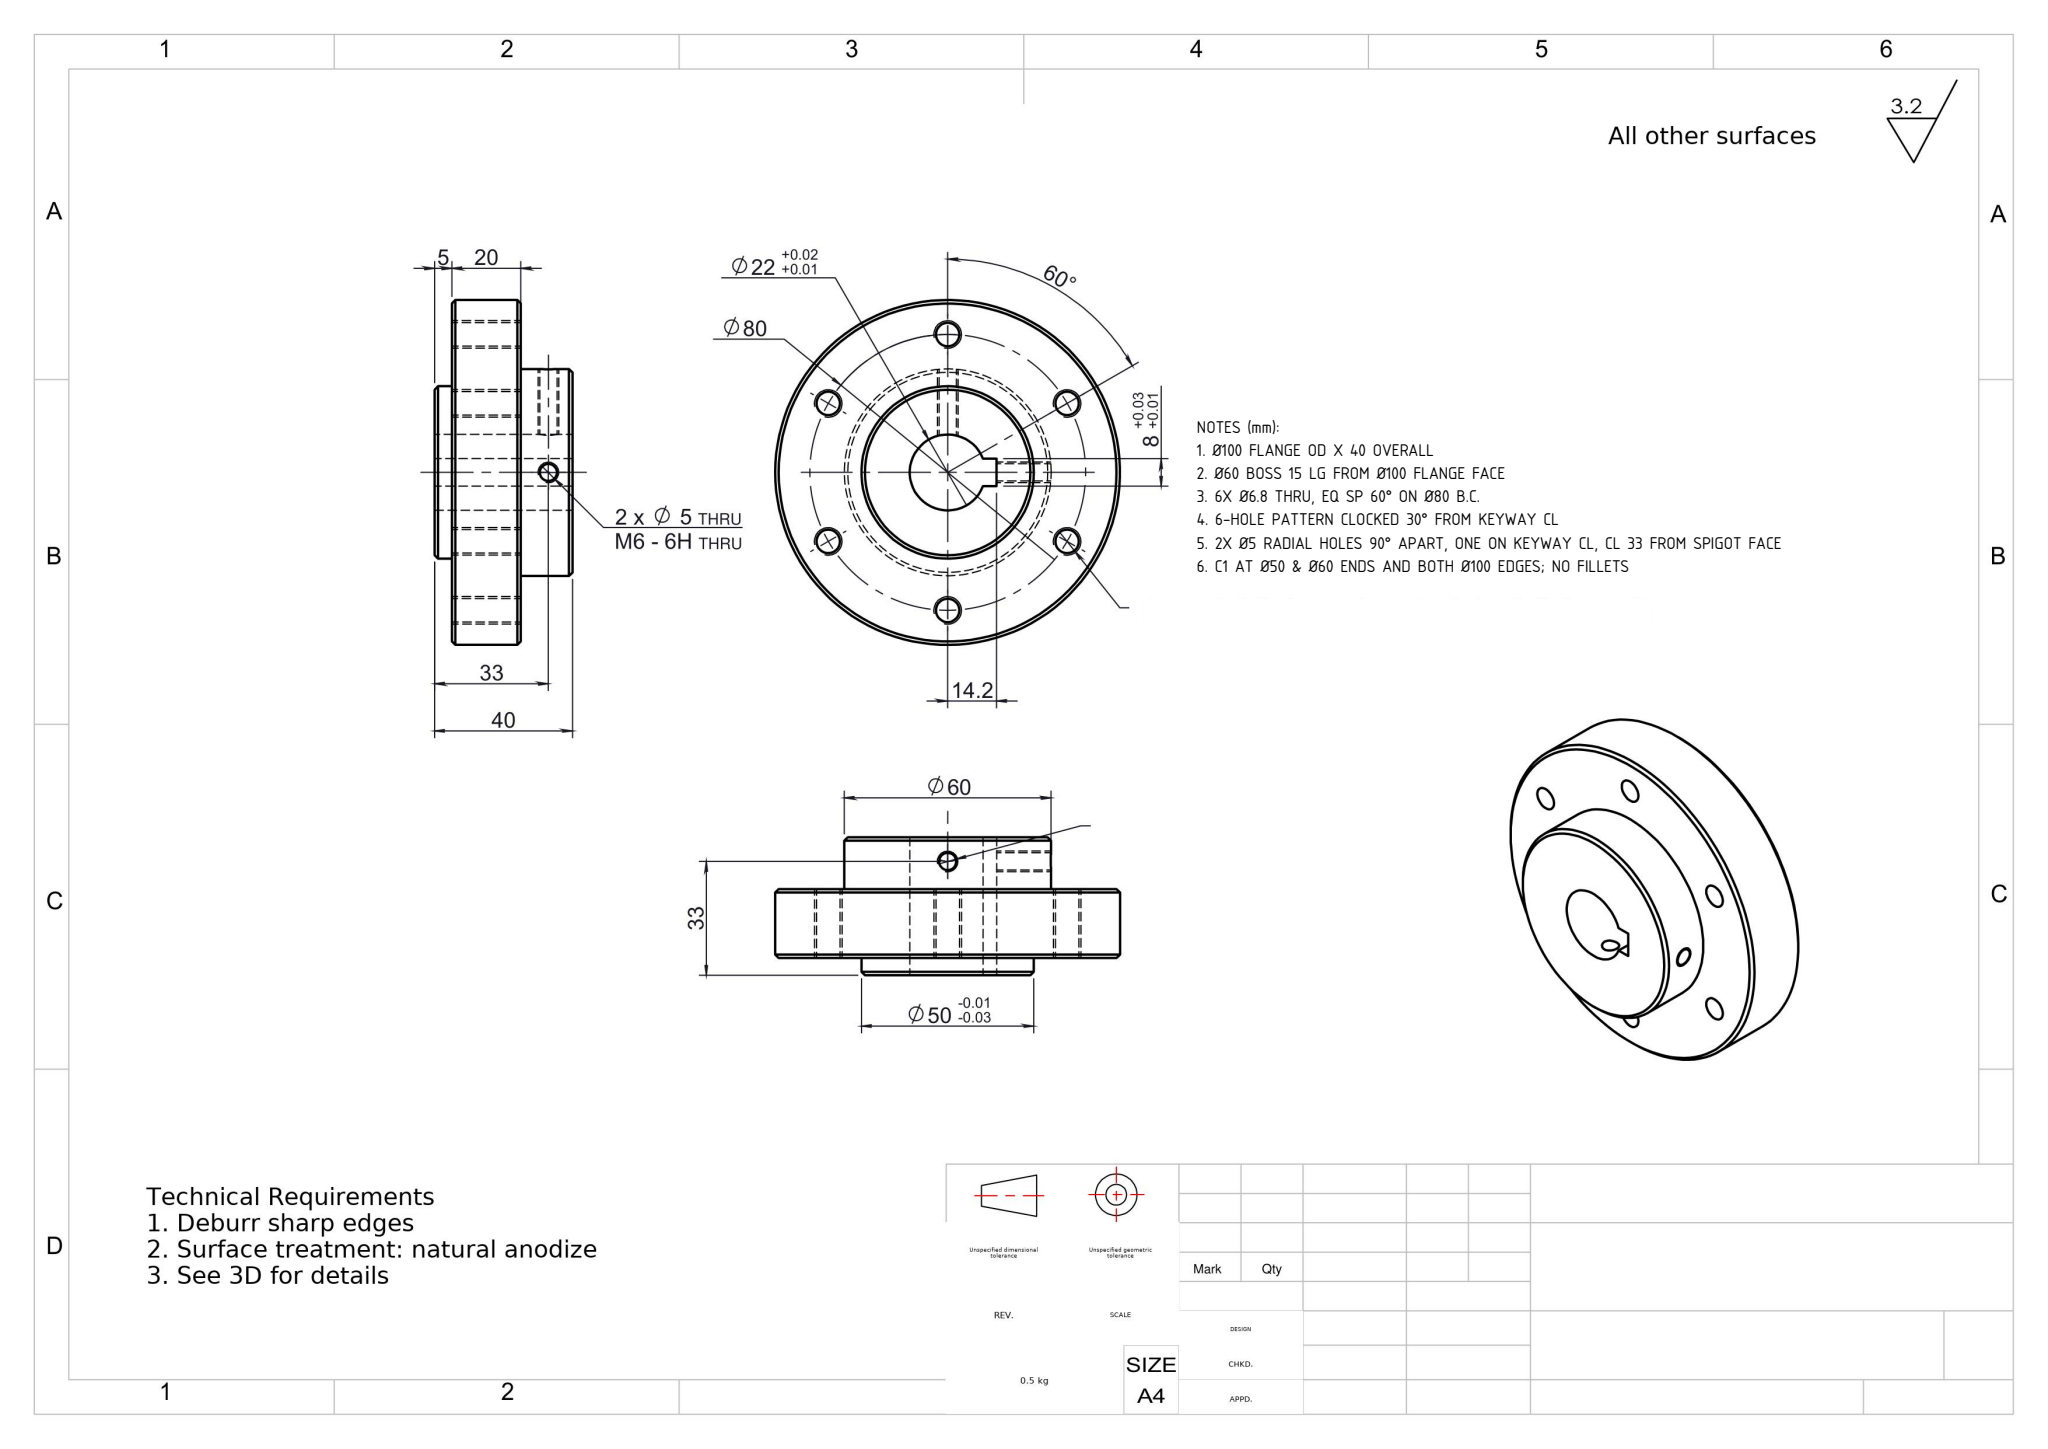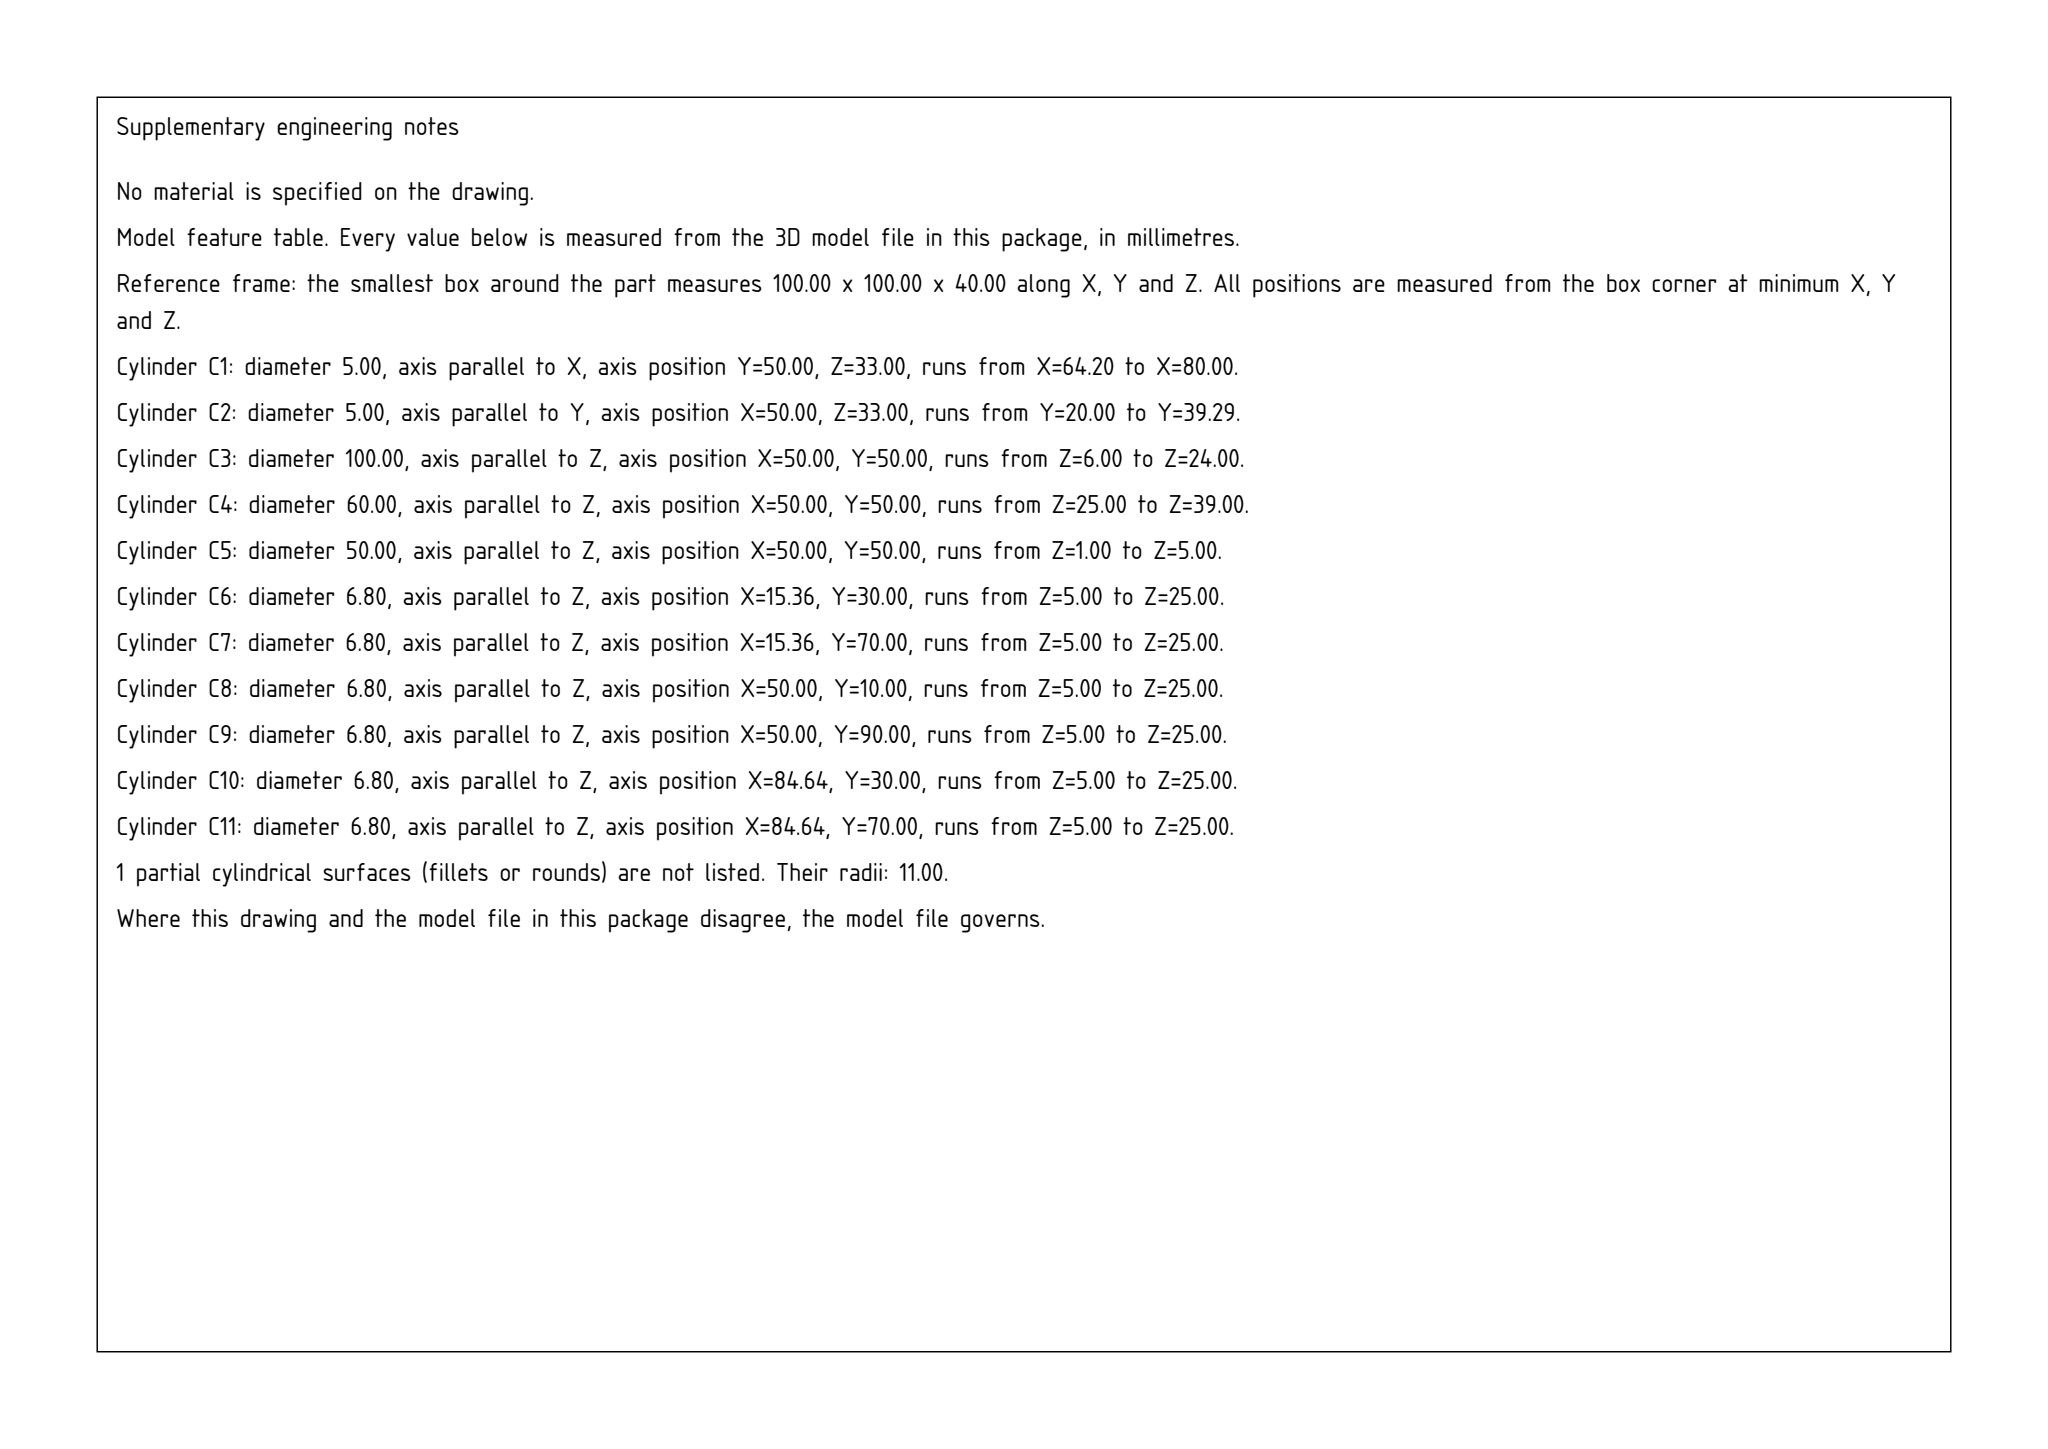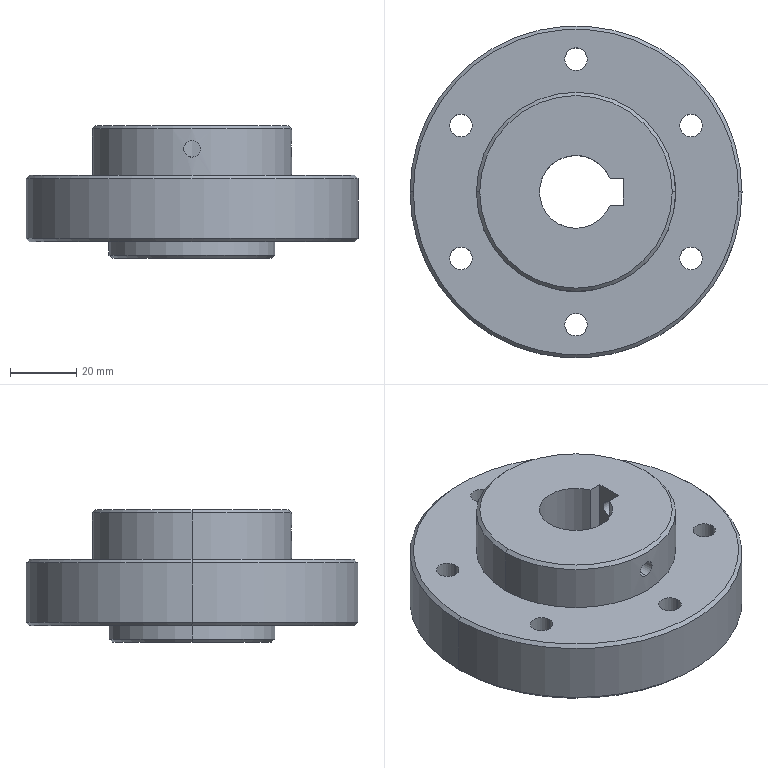Part | SolidWorks | mm | 1 solid | 38 faces | box 100 x 100 x 40 mm | volume 187475 mm3 | cylinder 23 | cone 8 | plane 7 | commonest cylinder face diameters 6.8 x12 5 x4 50 x2 60 x2 100 x2 22 x1
Drawing notes:
Ø100 FLANGE OD X 40 OVERALL | from the solid: Chamfer cones ref dia 98 at both flange edges -> Ø100 OD; bbox height 40 (z=0 to z=40)
Ø60 BOSS 15 LG FROM Ø100 FLANGE FACE | from the solid: Planes z=25 and z=40; Ø60 cyl L=14 plus 1 mm chamfer; bbox height 40
6X Ø6.8 THRU, EQ SP 60° ON Ø80 B.C. | from the solid: Six Ø6.8 z-axis holes at R40 from bore axis (50,50) -> Ø80 PCD, 60° apart
6-HOLE PATTERN CLOCKED 30° FROM KEYWAY CL | from the solid: Hole angles 30/90/150/210/270/330° from +X; keyway (y=46/54, x=64.2) on +X = 0°
2X Ø5 RADIAL HOLES 90° APART, ONE ON KEYWAY CL, CL 33 FROM SPIGOT FACE | from the solid: Ø5 x-axis (y=50) and y-axis (x=50) cylinders both at z=33; spigot end face z=0
C1 AT Ø50 & Ø60 ENDS AND BOTH Ø100 EDGES; NO FILLETS | from the solid: Cones 90° ref dia 98 (both flange edges), 48 (x2), 58 (x2) = 1 mm x 45°; no fillets
build123d program:
from build123d import *

# Parameters (mm, degrees)
SKETCH1_R              = 50
BOSS_EXTRUDE1_DEPTH    = 25
SKETCH2_R              = 30
BOSS_EXTRUDE2_DEPTH    = 15
SKETCH3_R              = 11
CUT_EXTRUDE1_DEPTH     = 82.24
SKETCH4_OUTSIDE_W      = 131.394
SKETCH4_OUTSIDE_H      = 131.394
SKETCH4_OUTSIDE_R      = 25
CUT_EXTRUDE2_DEPTH     = 5
SKETCH5_W              = 14.2
SKETCH5_H              = 8
CUT_EXTRUDE3_DEPTH     = 82.24
M8_TAPPED_HOLE1_D      = 6.8
CIRPATTERN1_COUNT      = 6
M6_TAPPED_HOLE1_REACH  = 104.47
M6_TAPPED_HOLE1_BORE_R = 2.5
CIRPATTERN2_COUNT      = 2
CIRPATTERN2_ANGLE      = 90
CHAMFER1_SIZE          = 1


with BuildPart() as part:
    # Sketch1 → Boss-Extrude1 (new body)
    with BuildSketch(Plane.XY):
        Circle(SKETCH1_R)
    extrude(amount=BOSS_EXTRUDE1_DEPTH)

    # Sketch2 → Boss-Extrude2 (add)
    with BuildSketch(Plane.XY.offset(25)):
        Circle(SKETCH2_R)
    extrude(amount=BOSS_EXTRUDE2_DEPTH)

    # Sketch3 → Cut-Extrude1 (cut, through all)
    with BuildSketch(Plane.XY.offset(40)):
        Circle(SKETCH3_R)
    extrude(amount=-CUT_EXTRUDE1_DEPTH, mode=Mode.SUBTRACT)

    # Sketch4 outside → Cut-Extrude2 (cut)
    with BuildSketch(Plane(origin=(0, 0, 0), x_dir=(-1, 0, 0), z_dir=(0, 0, -1))):
        Rectangle(SKETCH4_OUTSIDE_W, SKETCH4_OUTSIDE_H)
        Circle(SKETCH4_OUTSIDE_R, mode=Mode.SUBTRACT)
    extrude(amount=-CUT_EXTRUDE2_DEPTH, mode=Mode.SUBTRACT)

    # Sketch5 → Cut-Extrude3 (cut, through all)
    with BuildSketch(Plane(origin=(0, 0, 0), x_dir=(-1, 0, 0), z_dir=(0, 0, -1))):
        with Locations((-7.1, 0)):
            Rectangle(SKETCH5_W, SKETCH5_H)
    extrude(amount=-CUT_EXTRUDE3_DEPTH, mode=Mode.SUBTRACT)

    # M8 Tapped Hole1 (through all)
    with Locations(Plane(origin=(0, 0, 5), x_dir=(-1, 0, 0), z_dir=(0, 0, -1))):
        with Locations((0, 40)):
            m8_tapped_hole1 = Hole(M8_TAPPED_HOLE1_D / 2)

    # CirPattern1: M8 Tapped Hole1 ×6 about axis
    cirpattern1_axis = Axis((0, 0, 0), (0, 0, 1))
    for i in range(1, CIRPATTERN1_COUNT):
        add(m8_tapped_hole1.rotate(cirpattern1_axis, i * 360 / CIRPATTERN1_COUNT), mode=Mode.SUBTRACT)

    # M6 Tapped Hole1 bore → M6 Tapped Hole1 (cut, up to next)
    with BuildSketch(Plane(origin=(30, 0, 0), x_dir=(0, 0, -1), z_dir=(1, 0, 0)), mode=Mode.PRIVATE) as m6_tapped_hole1_sk1:
        with Locations((-33, 0)):
            Circle(M6_TAPPED_HOLE1_BORE_R)
    m6_tapped_hole1_tool1 = extrude(m6_tapped_hole1_sk1.sketch, amount=-M6_TAPPED_HOLE1_REACH, mode=Mode.PRIVATE) & part.part
    m6_tapped_hole1 = m6_tapped_hole1_tool1.solids().sort_by_distance((30, 0, 33))[0]
    add(m6_tapped_hole1, mode=Mode.SUBTRACT)

    # CirPattern2: M6 Tapped Hole1; each copy of M6 Tapped Hole1 runs up to whatever stops it at its own place
    cirpattern2_before = part.part  # the part as the pattern finds it: every copy runs up to it
    cirpattern2_m6_tapped_hole1_long = extrude(m6_tapped_hole1_sk1.sketch, amount=-M6_TAPPED_HOLE1_REACH, mode=Mode.PRIVATE)
    cirpattern2_m6_tapped_hole1_tool1 = cirpattern2_m6_tapped_hole1_long.rotate(Axis((0, 0, 40), (0, 0, -1)), 1 * CIRPATTERN2_ANGLE / (CIRPATTERN2_COUNT - 1)) & cirpattern2_before
    add(cirpattern2_m6_tapped_hole1_tool1.solids().sort_by_distance((0, -30, 33))[0], mode=Mode.SUBTRACT)

    # Chamfer1
    chamfer1_edges = [part.edges().sort_by_distance(p)[0] for p in [
        (-50, 0, 5),
        (25, 0, 0),
        (-50, 0, 25),
        (-30, 0, 40),
    ]]
    chamfer(chamfer1_edges, length=CHAMFER1_SIZE)


solid = part.part